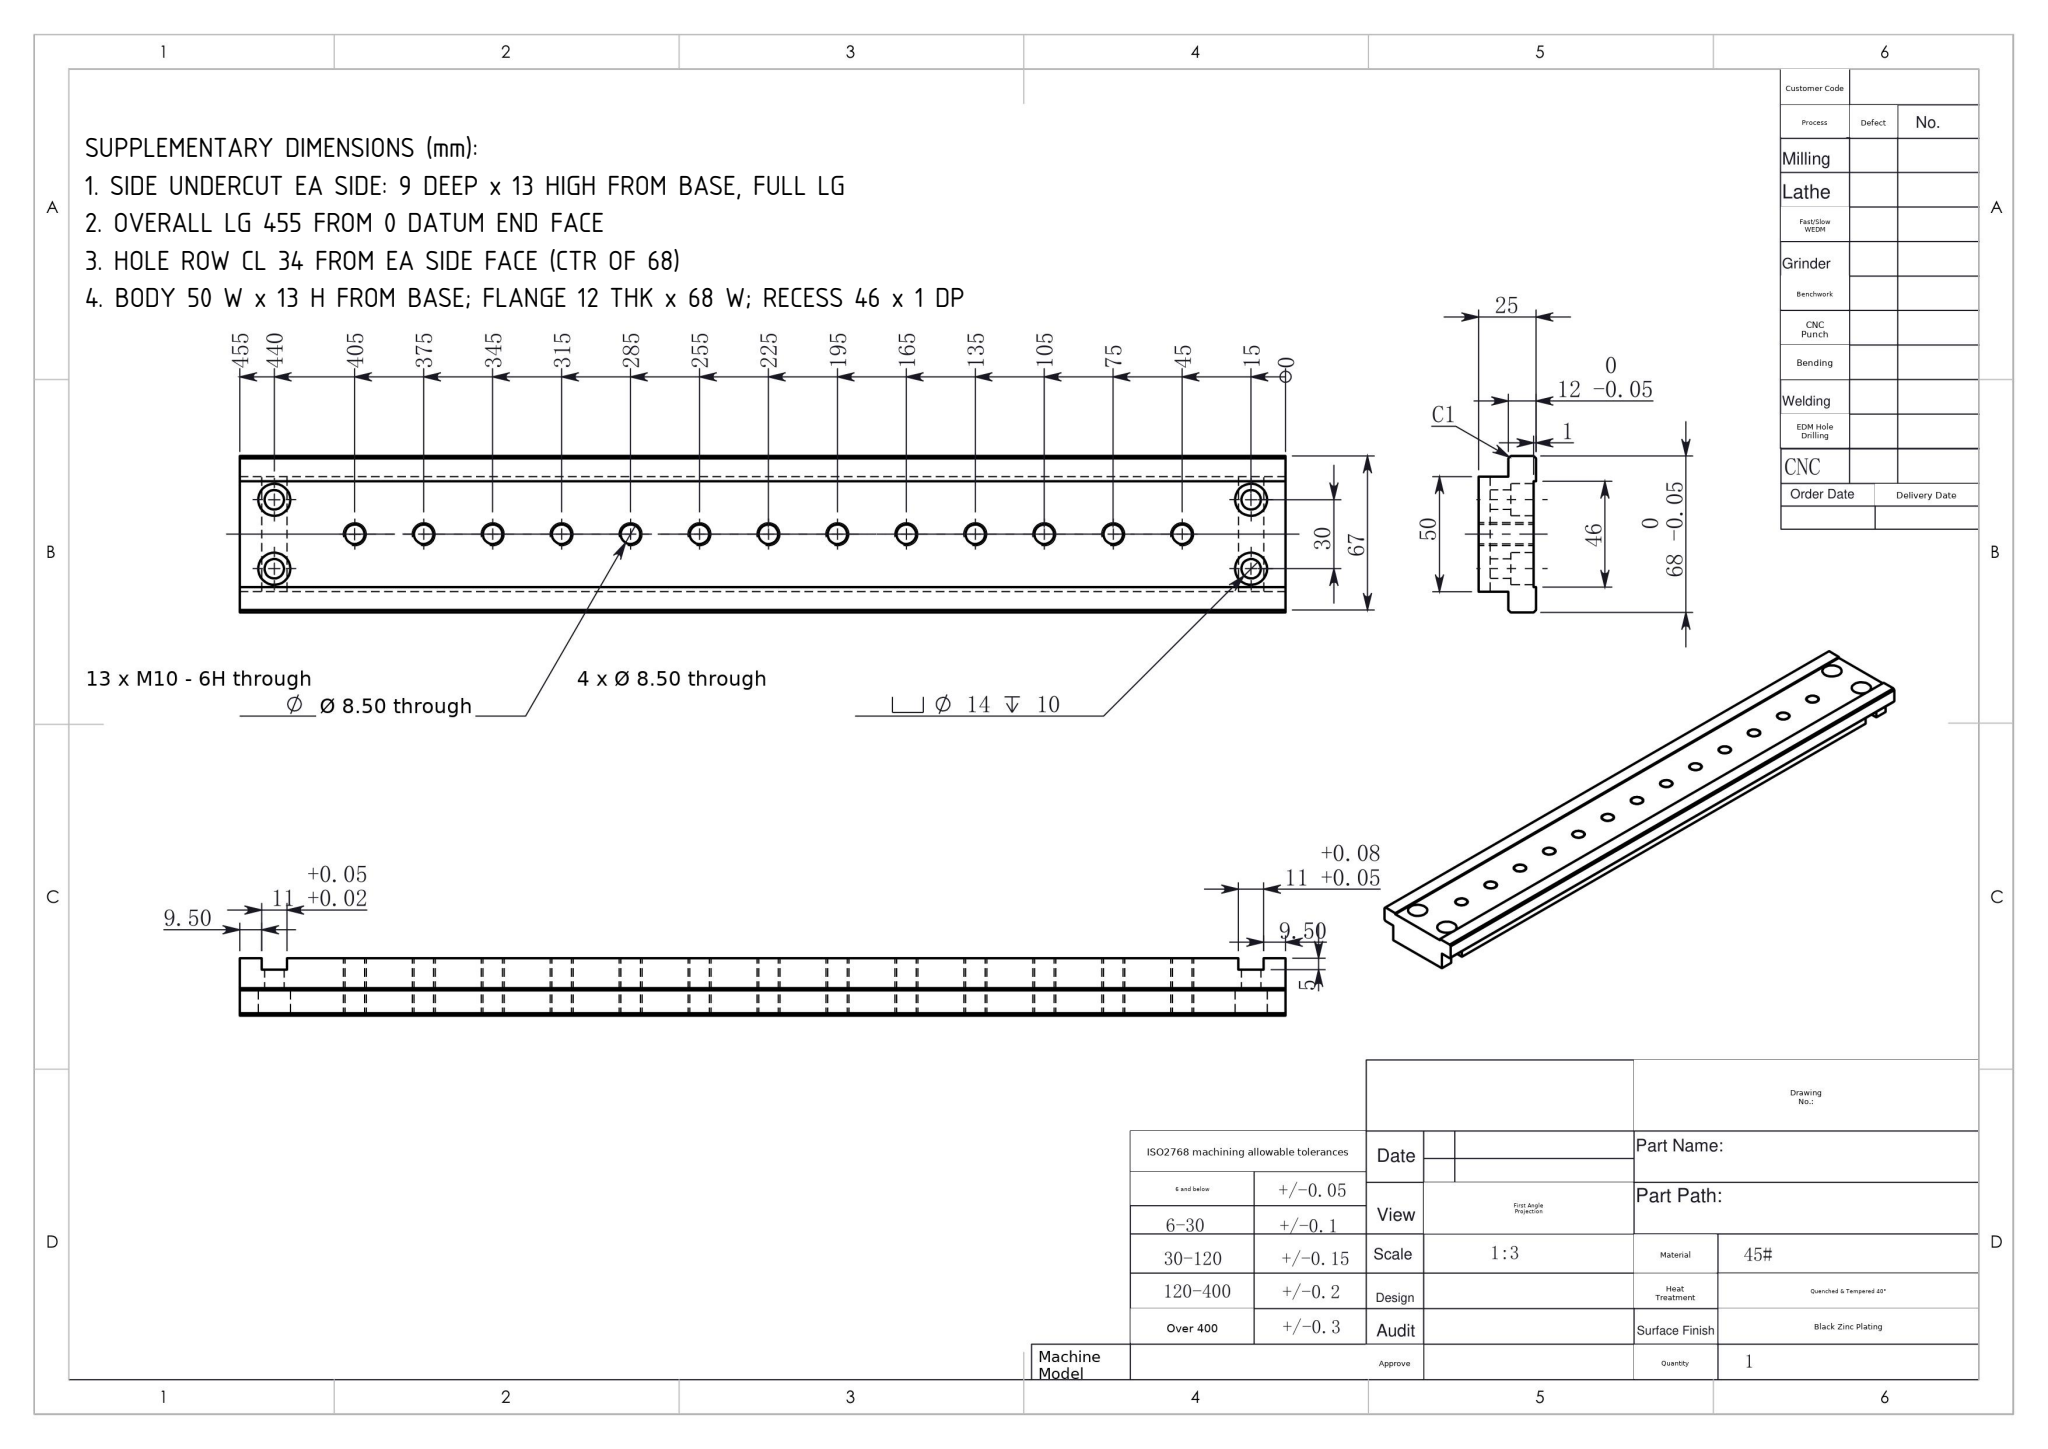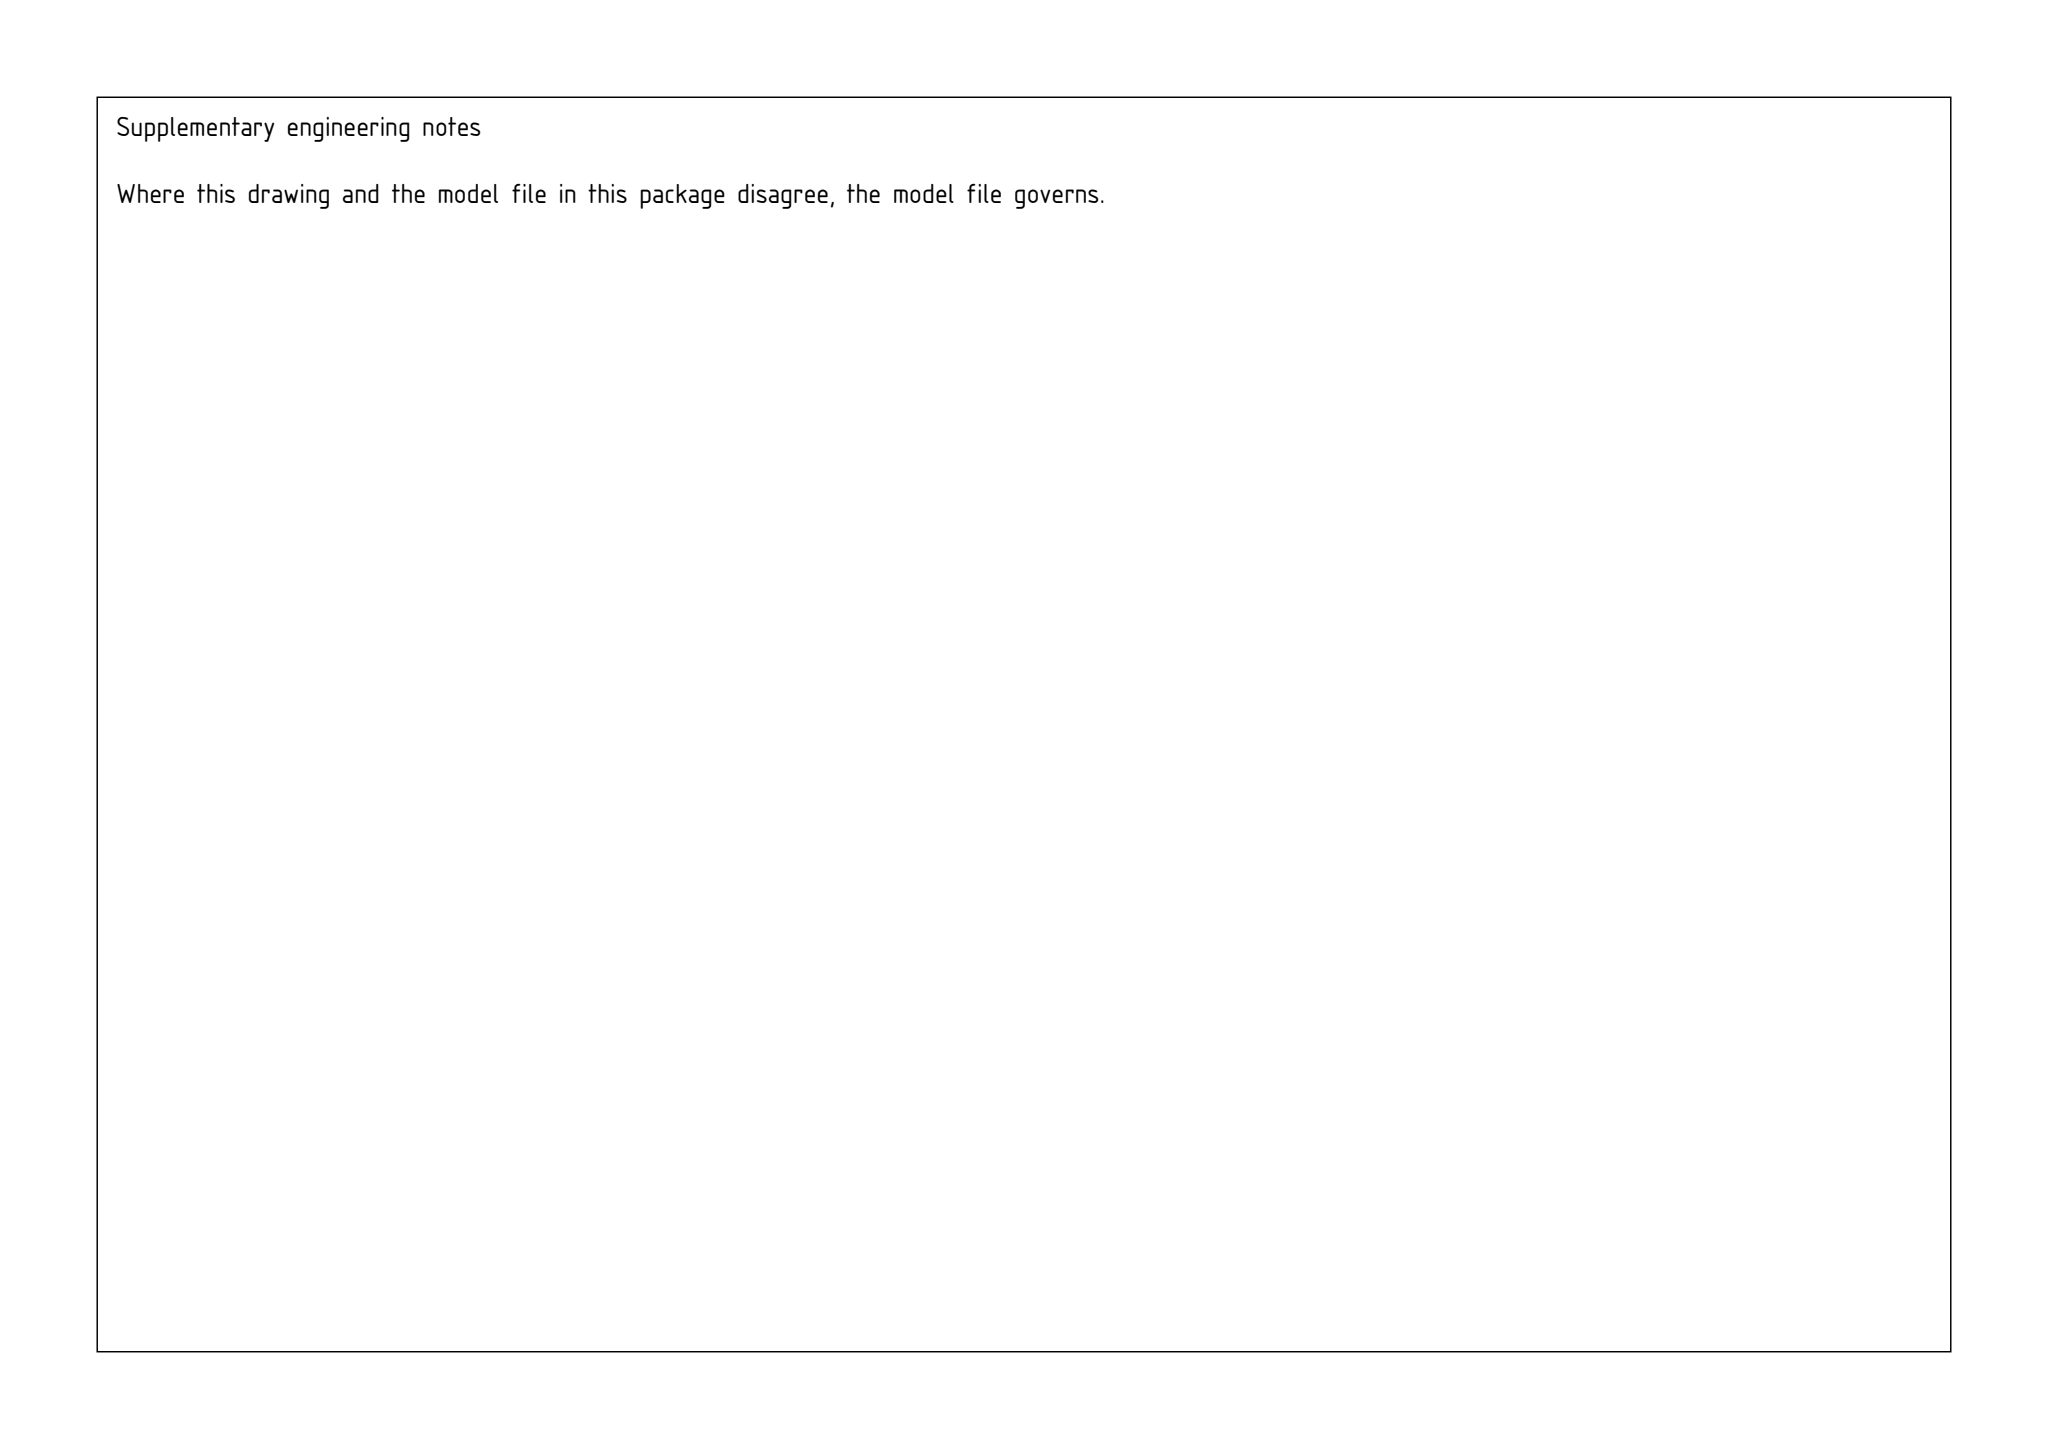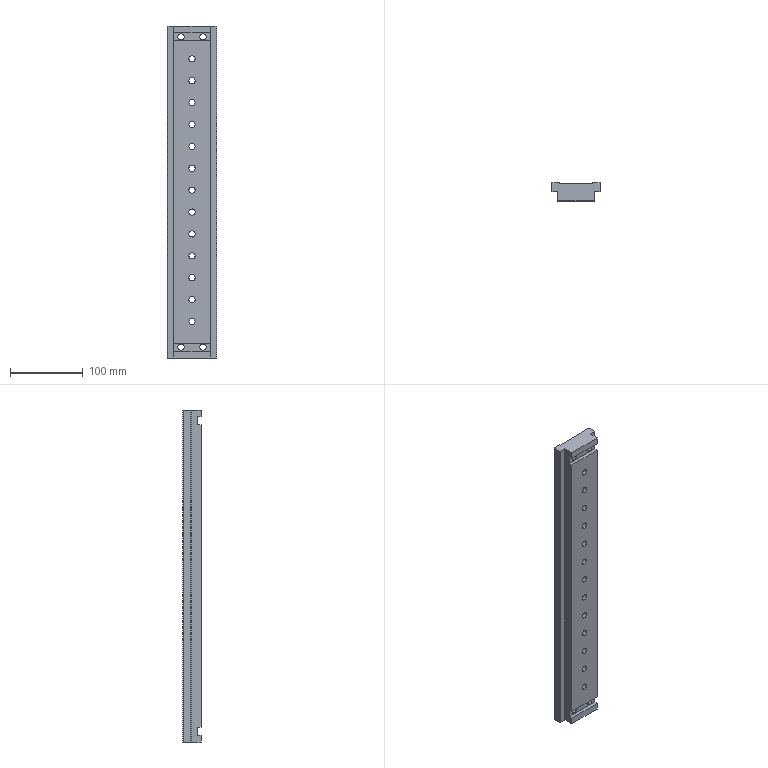Part | SolidWorks | mm | 1 solid | 72 faces | box 68 x 25 x 455 mm | volume 613785 mm3 | cylinder 42 | plane 30 | commonest cylinder face diameters 8.5 x34 14 x8
build123d program:
from build123d import *

# Parameters (mm, degrees)
BOSS_EXTRUDE1_DEPTH                                = 227.5
M10_TAPPED_HOLE1_D                                 = 8.5
SKETCH5_W                                          = 11
SKETCH5_H                                          = 14.831
CUT_EXTRUDE1_DEPTH                                 = 455
HOLE_SIZE_ACCORDING_TO_TYPE_1_OF_HEXAG_D           = 8.5
HOLE_SIZE_ACCORDING_TO_TYPE_1_OF_HEXAG_CBORE_D     = 14
HOLE_SIZE_ACCORDING_TO_TYPE_1_OF_HEXAG_CBORE_DEPTH = 10
CHAMFER1_SIZE                                      = 1


with BuildPart() as part:
    # Sketch2 → Boss-Extrude1 (new, symmetric)
    with BuildSketch(Plane.XY):
        Polygon((-34, 25), (-23, 25), (-23, 24), (23, 24), (23, 25), (34, 25), (34, 13), (25, 13), (25, 0), (-25, 0), (-25, 13), (-34, 13), align=None)
    extrude(amount=BOSS_EXTRUDE1_DEPTH, both=True)

    # M10 Tapped Hole1 (through all)
    with Locations(Plane(origin=(0, 24, 0), x_dir=(1, 0, 0), z_dir=(0, 1, 0))):
        with Locations((0, -182.5), (0, -152.5), (0, -122.5), (0, -92.5), (0, -62.5), (0, -32.5), (0, -2.5), (0, 27.5), (0, 57.5), (0, 87.5), (0, 117.5), (0, 147.5), (0, 177.5)):
            Hole(M10_TAPPED_HOLE1_D / 2)

    # Sketch5 → Cut-Extrude1 (cut)
    with BuildSketch(Plane(origin=(25, 0, 0), x_dir=(0, 0, -1), z_dir=(1, 0, 0))):
        with Locations((-212.5, -2.415)):
            Rectangle(SKETCH5_W, SKETCH5_H)
        with Locations((212.5, -2.415)):
            Rectangle(SKETCH5_W, SKETCH5_H)
    extrude(amount=-CUT_EXTRUDE1_DEPTH, mode=Mode.SUBTRACT)

    # Hole Size _according to_ Type 1 of Hexag (through all)
    with Locations(Plane(origin=(0, 24, 0), x_dir=(1, 0, 0), z_dir=(0, 1, 0))):
        with Locations((-15, -212.5), (15, -212.5), (15, 212.5), (-15, 212.5)):
            CounterBoreHole(HOLE_SIZE_ACCORDING_TO_TYPE_1_OF_HEXAG_D / 2, HOLE_SIZE_ACCORDING_TO_TYPE_1_OF_HEXAG_CBORE_D / 2, HOLE_SIZE_ACCORDING_TO_TYPE_1_OF_HEXAG_CBORE_DEPTH)

    # Chamfer1
    chamfer1_edges = [part.edges().sort_by_distance(p)[0] for p in [
        (34, 25, 0),
        (34, 13, 0),
        (-34, 13, 0),
        (-34, 25, 0),
    ]]
    chamfer(chamfer1_edges, length=CHAMFER1_SIZE)


solid = part.part